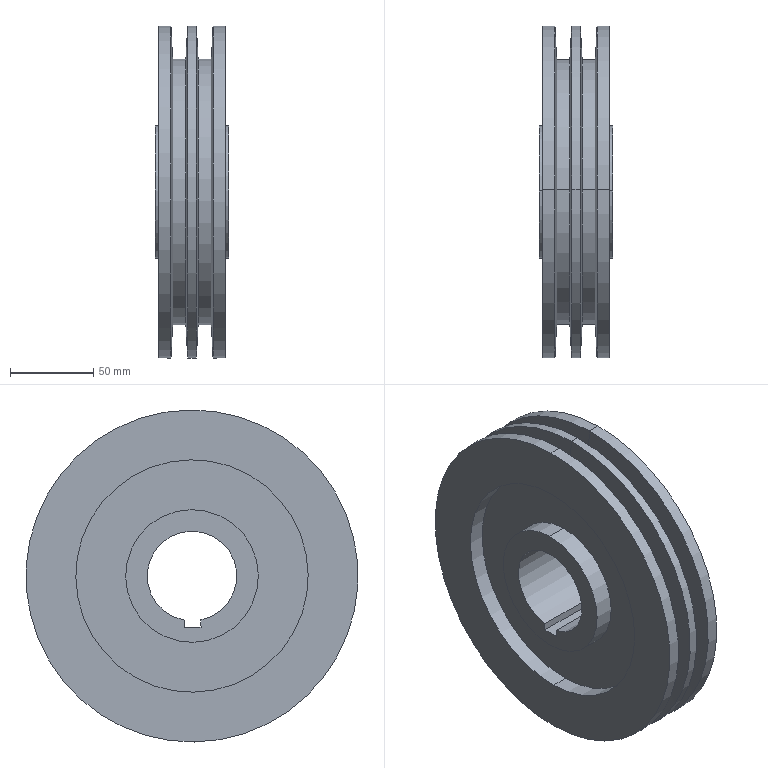Component | SolidWorks | Pulley1-1 | 1 solid | 37 faces | box 44 x 200 x 200 mm | volume 762387 mm3 | cylinder 20 | plane 9 | cone 8 | commonest cylinder face diameters 200 x6 160 x4 80 x4 140 x4 54 x2
build123d program:
from build123d import *

# Parameters (mm, degrees)
SKETCH1_5_R         = 100
SKETCH1_5_R_2       = 70
BOSS_EXTRUDE1_DEPTH = 20
SKETCH1_4_R         = 40
SKETCH1_4_R_2       = 27
BOSS_EXTRUDE2_DEPTH = 22
SKETCH1_5_2_R       = 70
SKETCH1_5_2_R_2     = 40
BOSS_EXTRUDE3_DEPTH = 10
SKETCH2_W           = 10
SKETCH2_H           = 8
CUT_EXTRUDE1_DEPTH  = 50


with BuildPart() as part:
    # Sketch1_5 → Boss-Extrude1 (new, symmetric)
    with BuildSketch(Plane(origin=(0, 0, 0), x_dir=(1, 0, 0), z_dir=(0, 1, 0))):
        with Locations(Location((0, 0, 0), (0, 0, 270))):
            Circle(SKETCH1_5_R)
        with Locations(Location((0, 0, 0), (0, 0, 270))):
            Circle(SKETCH1_5_R_2, mode=Mode.SUBTRACT)
    extrude(amount=BOSS_EXTRUDE1_DEPTH, both=True)



with BuildPart() as body_2:
    # Sketch1_4 → Boss-Extrude2 (new, symmetric)
    with BuildSketch(Plane(origin=(0, 0, 0), x_dir=(1, 0, 0), z_dir=(0, 1, 0))):
        with Locations(Location((0, 0, 0), (0, 0, 270))):
            Circle(SKETCH1_4_R)
        with Locations(Location((0, 0, 0), (0, 0, 270))):
            Circle(SKETCH1_4_R_2, mode=Mode.SUBTRACT)
    extrude(amount=BOSS_EXTRUDE2_DEPTH, both=True)


with BuildPart() as part_1:
    add(part.part)

    add(body_2.part)  # Boss-Extrude3 merges body 2
    # Sketch1_5 2 → Boss-Extrude3 (add, symmetric)
    with BuildSketch(Plane(origin=(0, 0, 0), x_dir=(1, 0, 0), z_dir=(0, 1, 0))):
        with Locations(Location((0, 0, 0), (0, 0, 270))):
            Circle(SKETCH1_5_2_R)
        with Locations(Location((0, 0, 0), (0, 0, 270))):
            Circle(SKETCH1_5_2_R_2, mode=Mode.SUBTRACT)
    extrude(amount=BOSS_EXTRUDE3_DEPTH, both=True)

    # Sketch2 → Cut-Extrude1 (cut)
    with BuildSketch(Plane.XZ.offset(22)):
        with Locations((0, 27)):
            Rectangle(SKETCH2_W, SKETCH2_H)
    extrude(amount=-CUT_EXTRUDE1_DEPTH, mode=Mode.SUBTRACT)

    # Sketch3 → Cut-Revolve1 (revolve, cut)
    with BuildSketch(Plane(origin=(0, 0, 0), x_dir=(0, 0, -1), z_dir=(1, 0, 0))):
        Polygon((-80, 7.676), (-80, 11.676), (-100, 12.676), (-100, 2.676), (-80, 3.676), align=None)
        Polygon((-80, -7.676), (-80, -11.676), (-100, -12.676), (-100, -2.676), (-80, -3.676), align=None)
    revolve(axis=Axis((0, 42.976, 0), (0, -1, 0)), mode=Mode.SUBTRACT)


solid = part_1.part

# Placed as in the assembly
solid = solid.moved(Location((141.571, -8.561, -165), (179.199, 0, -90)))
STEP:
#1=COLOUR_RGB('',0.7922,0.8196,0.9333);
#2=FILL_AREA_STYLE_COLOUR('',#1);
#3=FILL_AREA_STYLE('',(#2));
#4=SURFACE_STYLE_FILL_AREA(#3);
#5=SURFACE_SIDE_STYLE('',(#4));
#6=SURFACE_STYLE_USAGE(.BOTH.,#5);
#7=PRESENTATION_STYLE_ASSIGNMENT((#6));
#8=CARTESIAN_POINT('',(6.033,-0.3811,-9.645));
#9=VERTEX_POINT('',#8);
#10=CARTESIAN_POINT('',(6.033,-0.293,-3.347));
#11=VERTEX_POINT('',#10);
#12=CARTESIAN_POINT('',(6.033,-0.3371,-6.496));
#13=DIRECTION('',(-1.,-0.,-0.));
#14=DIRECTION('',(0.,-0.01398,-0.9999));
#15=AXIS2_PLACEMENT_3D('',#12,#13,#14);
#16=CIRCLE('',#15,3.15);
#17=EDGE_CURVE('',#9,#11,#16,.T.);
#18=ORIENTED_EDGE('',*,*,#17,.T.);
#19=CARTESIAN_POINT('',(5.718,-0.293,-3.347));
#20=VERTEX_POINT('',#19);
#21=CARTESIAN_POINT('',(3.882,-0.293,-3.347));
#22=DIRECTION('',(-1.,-0.,-0.));
#23=VECTOR('',#22,39.37);
#24=LINE('',#21,#23);
#25=EDGE_CURVE('',#11,#20,#24,.T.);
#26=ORIENTED_EDGE('',*,*,#25,.T.);
#27=CARTESIAN_POINT('',(5.718,-0.3811,-9.645));
#28=VERTEX_POINT('',#27);
#29=CARTESIAN_POINT('',(5.718,-0.3371,-6.496));
#30=DIRECTION('',(-1.,-0.,-0.));
#31=DIRECTION('',(0.,-0.01398,-0.9999));
#32=AXIS2_PLACEMENT_3D('',#29,#30,#31);
#33=CIRCLE('',#32,3.15);
#34=EDGE_CURVE('',#28,#20,#33,.T.);
#35=ORIENTED_EDGE('',*,*,#34,.F.);
#36=CARTESIAN_POINT('',(3.882,-0.3811,-9.645));
#37=DIRECTION('',(-1.,-0.,-0.));
#38=VECTOR('',#37,39.37);
#39=LINE('',#36,#38);
#40=EDGE_CURVE('',#9,#28,#39,.T.);
#41=ORIENTED_EDGE('',*,*,#40,.F.);
#42=EDGE_LOOP('',(#18,#26,#35,#41));
#43=FACE_OUTER_BOUND('',#42,.T.);
#44=CARTESIAN_POINT('',(3.882,-0.3371,-6.496));
#45=DIRECTION('',(-1.,-0.,-0.));
#46=DIRECTION('',(0.,-0.01398,-0.9999));
#47=AXIS2_PLACEMENT_3D('',#44,#45,#46);
#48=CYLINDRICAL_SURFACE('',#47,3.15);
#49=ADVANCED_FACE('',(#43),#48,.T.);
#50=ORIENTED_EDGE('',*,*,#17,.F.);
#51=CARTESIAN_POINT('',(6.073,-0.3921,-10.433));
#52=VERTEX_POINT('',#51);
#53=CARTESIAN_POINT('',(6.073,-0.3921,-10.433));
#54=DIRECTION('',(0.04994,-0.01396,-0.9987));
#55=VECTOR('',#54,39.37);
#56=LINE('',#53,#55);
#57=EDGE_CURVE('',#9,#52,#56,.T.);
#58=ORIENTED_EDGE('',*,*,#57,.T.);
#59=CARTESIAN_POINT('',(6.073,-0.282,-2.559));
#60=VERTEX_POINT('',#59);
#61=CARTESIAN_POINT('',(6.073,-0.3371,-6.496));
#62=DIRECTION('',(-1.,-0.,-0.));
#63=DIRECTION('',(0.,-0.01398,-0.9999));
#64=AXIS2_PLACEMENT_3D('',#61,#62,#63);
#65=CIRCLE('',#64,3.937);
#66=EDGE_CURVE('',#52,#60,#65,.T.);
#67=ORIENTED_EDGE('',*,*,#66,.T.);
#68=CARTESIAN_POINT('',(6.073,-0.282,-2.559));
#69=DIRECTION('',(0.04994,0.01396,0.9987));
#70=VECTOR('',#69,39.37);
#71=LINE('',#68,#70);
#72=EDGE_CURVE('',#11,#60,#71,.T.);
#73=ORIENTED_EDGE('',*,*,#72,.F.);
#74=EDGE_LOOP('',(#50,#58,#67,#73));
#75=FACE_OUTER_BOUND('',#74,.T.);
#76=CARTESIAN_POINT('',(6.073,-0.3371,-6.496));
#77=DIRECTION('',(1.,0.,0.));
#78=DIRECTION('',(0.,0.01398,0.9999));
#79=AXIS2_PLACEMENT_3D('',#76,#77,#78);
#80=CONICAL_SURFACE('',#79,3.937,1.521);
#81=ADVANCED_FACE('',(#75),#80,.T.);
#82=ORIENTED_EDGE('',*,*,#34,.T.);
#83=CARTESIAN_POINT('',(5.679,-0.282,-2.559));
#84=VERTEX_POINT('',#83);
#85=CARTESIAN_POINT('',(5.718,-0.293,-3.347));
#86=DIRECTION('',(-0.04994,0.01396,0.9987));
#87=VECTOR('',#86,39.37);
#88=LINE('',#85,#87);
#89=EDGE_CURVE('',#20,#84,#88,.T.);
#90=ORIENTED_EDGE('',*,*,#89,.T.);
#91=CARTESIAN_POINT('',(5.679,-0.3921,-10.433));
#92=VERTEX_POINT('',#91);
#93=CARTESIAN_POINT('',(5.679,-0.3371,-6.496));
#94=DIRECTION('',(-1.,-0.,-0.));
#95=DIRECTION('',(0.,-0.01398,-0.9999));
#96=AXIS2_PLACEMENT_3D('',#93,#94,#95);
#97=CIRCLE('',#96,3.937);
#98=EDGE_CURVE('',#92,#84,#97,.T.);
#99=ORIENTED_EDGE('',*,*,#98,.F.);
#100=CARTESIAN_POINT('',(5.718,-0.3811,-9.645));
#101=DIRECTION('',(-0.04994,-0.01396,-0.9987));
#102=VECTOR('',#101,39.37);
#103=LINE('',#100,#102);
#104=EDGE_CURVE('',#28,#92,#103,.T.);
#105=ORIENTED_EDGE('',*,*,#104,.F.);
#106=EDGE_LOOP('',(#82,#90,#99,#105));
#107=FACE_OUTER_BOUND('',#106,.T.);
#108=CARTESIAN_POINT('',(5.718,-0.3371,-6.496));
#109=DIRECTION('',(-1.,-0.,-0.));
#110=DIRECTION('',(0.,-0.01398,-0.9999));
#111=AXIS2_PLACEMENT_3D('',#108,#109,#110);
#112=CONICAL_SURFACE('',#111,3.15,1.521);
#113=ADVANCED_FACE('',(#107),#112,.T.);
#114=CARTESIAN_POINT('',(5.429,-0.3811,-9.645));
#115=VERTEX_POINT('',#114);
#116=CARTESIAN_POINT('',(5.429,-0.293,-3.347));
#117=VERTEX_POINT('',#116);
#118=CARTESIAN_POINT('',(5.429,-0.3371,-6.496));
#119=DIRECTION('',(-1.,-0.,-0.));
#120=DIRECTION('',(0.,-0.01398,-0.9999));
#121=AXIS2_PLACEMENT_3D('',#118,#119,#120);
#122=CIRCLE('',#121,3.15);
#123=EDGE_CURVE('',#115,#117,#122,.T.);
#124=ORIENTED_EDGE('',*,*,#123,.F.);
#125=CARTESIAN_POINT('',(5.468,-0.3921,-10.433));
#126=VERTEX_POINT('',#125);
#127=CARTESIAN_POINT('',(5.468,-0.3921,-10.433));
#128=DIRECTION('',(0.04994,-0.01396,-0.9987));
#129=VECTOR('',#128,39.37);
#130=LINE('',#127,#129);
#131=EDGE_CURVE('',#115,#126,#130,.T.);
#132=ORIENTED_EDGE('',*,*,#131,.T.);
#133=CARTESIAN_POINT('',(5.468,-0.282,-2.559));
#134=VERTEX_POINT('',#133);
#135=CARTESIAN_POINT('',(5.468,-0.3371,-6.496));
#136=DIRECTION('',(-1.,-0.,-0.));
#137=DIRECTION('',(0.,-0.01398,-0.9999));
#138=AXIS2_PLACEMENT_3D('',#135,#136,#137);
#139=CIRCLE('',#138,3.937);
#140=EDGE_CURVE('',#126,#134,#139,.T.);
#141=ORIENTED_EDGE('',*,*,#140,.T.);
#142=CARTESIAN_POINT('',(5.468,-0.282,-2.559));
#143=DIRECTION('',(0.04994,0.01396,0.9987));
#144=VECTOR('',#143,39.37);
#145=LINE('',#142,#144);
#146=EDGE_CURVE('',#117,#134,#145,.T.);
#147=ORIENTED_EDGE('',*,*,#146,.F.);
#148=EDGE_LOOP('',(#124,#132,#141,#147));
#149=FACE_OUTER_BOUND('',#148,.T.);
#150=CARTESIAN_POINT('',(5.468,-0.3371,-6.496));
#151=DIRECTION('',(1.,0.,0.));
#152=DIRECTION('',(0.,0.01398,0.9999));
#153=AXIS2_PLACEMENT_3D('',#150,#151,#152);
#154=CONICAL_SURFACE('',#153,3.937,1.521);
#155=ADVANCED_FACE('',(#149),#154,.T.);
#156=ORIENTED_EDGE('',*,*,#123,.T.);
#157=CARTESIAN_POINT('',(5.114,-0.293,-3.347));
#158=VERTEX_POINT('',#157);
#159=CARTESIAN_POINT('',(3.882,-0.293,-3.347));
#160=DIRECTION('',(-1.,-0.,-0.));
#161=VECTOR('',#160,39.37);
#162=LINE('',#159,#161);
#163=EDGE_CURVE('',#117,#158,#162,.T.);
#164=ORIENTED_EDGE('',*,*,#163,.T.);
#165=CARTESIAN_POINT('',(5.114,-0.3811,-9.645));
#166=VERTEX_POINT('',#165);
#167=CARTESIAN_POINT('',(5.114,-0.3371,-6.496));
#168=DIRECTION('',(-1.,-0.,-0.));
#169=DIRECTION('',(0.,-0.01398,-0.9999));
#170=AXIS2_PLACEMENT_3D('',#167,#168,#169);
#171=CIRCLE('',#170,3.15);
#172=EDGE_CURVE('',#166,#158,#171,.T.);
#173=ORIENTED_EDGE('',*,*,#172,.F.);
#174=CARTESIAN_POINT('',(3.882,-0.3811,-9.645));
#175=DIRECTION('',(-1.,-0.,-0.));
#176=VECTOR('',#175,39.37);
#177=LINE('',#174,#176);
#178=EDGE_CURVE('',#115,#166,#177,.T.);
#179=ORIENTED_EDGE('',*,*,#178,.F.);
#180=EDGE_LOOP('',(#156,#164,#173,#179));
#181=FACE_OUTER_BOUND('',#180,.T.);
#182=CARTESIAN_POINT('',(3.882,-0.3371,-6.496));
#183=DIRECTION('',(-1.,-0.,-0.));
#184=DIRECTION('',(0.,-0.01398,-0.9999));
#185=AXIS2_PLACEMENT_3D('',#182,#183,#184);
#186=CYLINDRICAL_SURFACE('',#185,3.15);
#187=ADVANCED_FACE('',(#181),#186,.T.);
#188=ORIENTED_EDGE('',*,*,#172,.T.);
#189=CARTESIAN_POINT('',(5.075,-0.282,-2.559));
#190=VERTEX_POINT('',#189);
#191=CARTESIAN_POINT('',(5.114,-0.293,-3.347));
#192=DIRECTION('',(-0.04994,0.01396,0.9987));
#193=VECTOR('',#192,39.37);
#194=LINE('',#191,#193);
#195=EDGE_CURVE('',#158,#190,#194,.T.);
#196=ORIENTED_EDGE('',*,*,#195,.T.);
#197=CARTESIAN_POINT('',(5.075,-0.3921,-10.433));
#198=VERTEX_POINT('',#197);
#199=CARTESIAN_POINT('',(5.075,-0.3371,-6.496));
#200=DIRECTION('',(-1.,-0.,-0.));
#201=DIRECTION('',(0.,-0.01398,-0.9999));
#202=AXIS2_PLACEMENT_3D('',#199,#200,#201);
#203=CIRCLE('',#202,3.937);
#204=EDGE_CURVE('',#198,#190,#203,.T.);
#205=ORIENTED_EDGE('',*,*,#204,.F.);
#206=CARTESIAN_POINT('',(5.114,-0.3811,-9.645));
#207=DIRECTION('',(-0.04994,-0.01396,-0.9987));
#208=VECTOR('',#207,39.37);
#209=LINE('',#206,#208);
#210=EDGE_CURVE('',#166,#198,#209,.T.);
#211=ORIENTED_EDGE('',*,*,#210,.F.);
#212=EDGE_LOOP('',(#188,#196,#205,#211));
#213=FACE_OUTER_BOUND('',#212,.T.);
#214=CARTESIAN_POINT('',(5.114,-0.3371,-6.496));
#215=DIRECTION('',(-1.,-0.,-0.));
#216=DIRECTION('',(0.,-0.01398,-0.9999));
#217=AXIS2_PLACEMENT_3D('',#214,#215,#216);
#218=CONICAL_SURFACE('',#217,3.15,1.521);
#219=ADVANCED_FACE('',(#213),#218,.T.);
#220=CARTESIAN_POINT('',(4.708,-0.3591,-8.071));
#221=VERTEX_POINT('',#220);
#222=CARTESIAN_POINT('',(4.708,-0.315,-4.921));
#223=VERTEX_POINT('',#222);
#224=CARTESIAN_POINT('',(4.708,-0.3371,-6.496));
#225=DIRECTION('',(-1.,-0.,-0.));
#226=DIRECTION('',(0.,-0.01398,-0.9999));
#227=AXIS2_PLACEMENT_3D('',#224,#225,#226);
#228=CIRCLE('',#227,1.575);
#229=EDGE_CURVE('',#221,#223,#228,.T.);
#230=ORIENTED_EDGE('',*,*,#229,.F.);
#231=CARTESIAN_POINT('',(5.18,-0.3591,-8.071));
#232=VERTEX_POINT('',#231);
#233=CARTESIAN_POINT('',(4.708,-0.3591,-8.071));
#234=DIRECTION('',(1.,0.,0.));
#235=VECTOR('',#234,39.37);
#236=LINE('',#233,#235);
#237=EDGE_CURVE('',#221,#232,#236,.T.);
#238=ORIENTED_EDGE('',*,*,#237,.T.);
#239=CARTESIAN_POINT('',(5.18,-0.315,-4.921));
#240=VERTEX_POINT('',#239);
#241=CARTESIAN_POINT('',(5.18,-0.3371,-6.496));
#242=DIRECTION('',(-1.,-0.,-0.));
#243=DIRECTION('',(0.,-0.01398,-0.9999));
#244=AXIS2_PLACEMENT_3D('',#241,#242,#243);
#245=CIRCLE('',#244,1.575);
#246=EDGE_CURVE('',#232,#240,#245,.T.);
#247=ORIENTED_EDGE('',*,*,#246,.T.);
#248=CARTESIAN_POINT('',(4.708,-0.315,-4.921));
#249=DIRECTION('',(1.,0.,0.));
#250=VECTOR('',#249,39.37);
#251=LINE('',#248,#250);
#252=EDGE_CURVE('',#223,#240,#251,.T.);
#253=ORIENTED_EDGE('',*,*,#252,.F.);
#254=EDGE_LOOP('',(#230,#238,#247,#253));
#255=FACE_OUTER_BOUND('',#254,.T.);
#256=CARTESIAN_POINT('',(4.708,-0.3371,-6.496));
#257=DIRECTION('',(1.,0.,0.));
#258=DIRECTION('',(0.,0.01398,0.9999));
#259=AXIS2_PLACEMENT_3D('',#256,#257,#258);
#260=CYLINDRICAL_SURFACE('',#259,1.575);
#261=ADVANCED_FACE('',(#255),#260,.T.);
#262=CARTESIAN_POINT('',(4.708,-0.5485,-7.538));
#263=VERTEX_POINT('',#262);
#264=CARTESIAN_POINT('',(4.708,-0.3222,-5.433));
#265=VERTEX_POINT('',#264);
#266=CARTESIAN_POINT('',(4.708,-0.3371,-6.496));
#267=DIRECTION('',(-1.,-0.,-0.));
#268=DIRECTION('',(0.,-0.01398,-0.9999));
#269=AXIS2_PLACEMENT_3D('',#266,#267,#268);
#270=CIRCLE('',#269,1.063);
#271=EDGE_CURVE('',#263,#265,#270,.T.);
#272=ORIENTED_EDGE('',*,*,#271,.T.);
#273=CARTESIAN_POINT('',(6.44,-0.3222,-5.433));
#274=VERTEX_POINT('',#273);
#275=CARTESIAN_POINT('',(4.708,-0.3222,-5.433));
#276=DIRECTION('',(1.,0.,0.));
#277=VECTOR('',#276,39.37);
#278=LINE('',#275,#277);
#279=EDGE_CURVE('',#265,#274,#278,.T.);
#280=ORIENTED_EDGE('',*,*,#279,.T.);
#281=CARTESIAN_POINT('',(6.44,-0.5485,-7.538));
#282=VERTEX_POINT('',#281);
#283=CARTESIAN_POINT('',(6.44,-0.3371,-6.496));
#284=DIRECTION('',(-1.,-0.,-0.));
#285=DIRECTION('',(0.,-0.01398,-0.9999));
#286=AXIS2_PLACEMENT_3D('',#283,#284,#285);
#287=CIRCLE('',#286,1.063);
#288=EDGE_CURVE('',#282,#274,#287,.T.);
#289=ORIENTED_EDGE('',*,*,#288,.F.);
#290=CARTESIAN_POINT('',(4.708,-0.5485,-7.538));
#291=DIRECTION('',(1.,0.,0.));
#292=VECTOR('',#291,39.37);
#293=LINE('',#290,#292);
#294=EDGE_CURVE('',#263,#282,#293,.T.);
#295=ORIENTED_EDGE('',*,*,#294,.F.);
#296=EDGE_LOOP('',(#272,#280,#289,#295));
#297=FACE_OUTER_BOUND('',#296,.T.);
#298=CARTESIAN_POINT('',(4.708,-0.3371,-6.496));
#299=DIRECTION('',(1.,0.,0.));
#300=DIRECTION('',(0.,0.01398,0.9999));
#301=AXIS2_PLACEMENT_3D('',#298,#299,#300);
#302=CYLINDRICAL_SURFACE('',#301,1.063);
#303=ADVANCED_FACE('',(#297),#302,.F.);
#304=CARTESIAN_POINT('',(5.967,-0.315,-4.921));
#305=VERTEX_POINT('',#304);
#306=CARTESIAN_POINT('',(5.967,-0.3591,-8.071));
#307=VERTEX_POINT('',#306);
#308=CARTESIAN_POINT('',(5.967,-0.3371,-6.496));
#309=DIRECTION('',(1.,0.,0.));
#310=DIRECTION('',(0.,-0.01398,-0.9999));
#311=AXIS2_PLACEMENT_3D('',#308,#309,#310);
#312=CIRCLE('',#311,1.575);
#313=EDGE_CURVE('',#305,#307,#312,.T.);
#314=ORIENTED_EDGE('',*,*,#313,.T.);
#315=CARTESIAN_POINT('',(6.44,-0.3591,-8.071));
#316=VERTEX_POINT('',#315);
#317=CARTESIAN_POINT('',(4.708,-0.3591,-8.071));
#318=DIRECTION('',(1.,0.,0.));
#319=VECTOR('',#318,39.37);
#320=LINE('',#317,#319);
#321=EDGE_CURVE('',#307,#316,#320,.T.);
#322=ORIENTED_EDGE('',*,*,#321,.T.);
#323=CARTESIAN_POINT('',(6.44,-0.315,-4.921));
#324=VERTEX_POINT('',#323);
#325=CARTESIAN_POINT('',(6.44,-0.3371,-6.496));
#326=DIRECTION('',(-1.,-0.,-0.));
#327=DIRECTION('',(0.,-0.01398,-0.9999));
#328=AXIS2_PLACEMENT_3D('',#325,#326,#327);
#329=CIRCLE('',#328,1.575);
#330=EDGE_CURVE('',#316,#324,#329,.T.);
#331=ORIENTED_EDGE('',*,*,#330,.T.);
#332=CARTESIAN_POINT('',(4.708,-0.315,-4.921));
#333=DIRECTION('',(1.,0.,0.));
#334=VECTOR('',#333,39.37);
#335=LINE('',#332,#334);
#336=EDGE_CURVE('',#305,#324,#335,.T.);
#337=ORIENTED_EDGE('',*,*,#336,.F.);
#338=EDGE_LOOP('',(#314,#322,#331,#337));
#339=FACE_OUTER_BOUND('',#338,.T.);
#340=CARTESIAN_POINT('',(4.708,-0.3371,-6.496));
#341=DIRECTION('',(1.,0.,0.));
#342=DIRECTION('',(0.,0.01398,0.9999));
#343=AXIS2_PLACEMENT_3D('',#340,#341,#342);
#344=CYLINDRICAL_SURFACE('',#343,1.575);
#345=ADVANCED_FACE('',(#339),#344,.T.);
#346=ORIENTED_EDGE('',*,*,#66,.F.);
#347=CARTESIAN_POINT('',(6.361,-0.3921,-10.433));
#348=VERTEX_POINT('',#347);
#349=CARTESIAN_POINT('',(4.786,-0.3921,-10.433));
#350=DIRECTION('',(1.,0.,0.));
#351=VECTOR('',#350,39.37);
#352=LINE('',#349,#351);
#353=EDGE_CURVE('',#52,#348,#352,.T.);
#354=ORIENTED_EDGE('',*,*,#353,.T.);
#355=CARTESIAN_POINT('',(6.361,-0.282,-2.559));
#356=VERTEX_POINT('',#355);
#357=CARTESIAN_POINT('',(6.361,-0.3371,-6.496));
#358=DIRECTION('',(-1.,-0.,-0.));
#359=DIRECTION('',(0.,-0.01398,-0.9999));
#360=AXIS2_PLACEMENT_3D('',#357,#358,#359);
#361=CIRCLE('',#360,3.937);
#362=EDGE_CURVE('',#348,#356,#361,.T.);
#363=ORIENTED_EDGE('',*,*,#362,.T.);
#364=CARTESIAN_POINT('',(4.786,-0.282,-2.559));
#365=DIRECTION('',(1.,0.,0.));
#366=VECTOR('',#365,39.37);
#367=LINE('',#364,#366);
#368=EDGE_CURVE('',#60,#356,#367,.T.);
#369=ORIENTED_EDGE('',*,*,#368,.F.);
#370=EDGE_LOOP('',(#346,#354,#363,#369));
#371=FACE_OUTER_BOUND('',#370,.T.);
#372=CARTESIAN_POINT('',(4.786,-0.3371,-6.496));
#373=DIRECTION('',(1.,0.,0.));
#374=DIRECTION('',(-0.,0.01398,0.9999));
#375=AXIS2_PLACEMENT_3D('',#372,#373,#374);
#376=CYLINDRICAL_SURFACE('',#375,3.937);
#377=ADVANCED_FACE('',(#371),#376,.T.);
#378=CARTESIAN_POINT('',(4.786,-0.2985,-3.74));
#379=VERTEX_POINT('',#378);
#380=CARTESIAN_POINT('',(4.786,-0.3756,-9.252));
#381=VERTEX_POINT('',#380);
#382=CARTESIAN_POINT('',(4.786,-0.3371,-6.496));
#383=DIRECTION('',(-1.,-0.,-0.));
#384=DIRECTION('',(0.,-0.01398,-0.9999));
#385=AXIS2_PLACEMENT_3D('',#382,#383,#384);
#386=CIRCLE('',#385,2.756);
#387=EDGE_CURVE('',#379,#381,#386,.T.);
#388=ORIENTED_EDGE('',*,*,#387,.T.);
#389=CARTESIAN_POINT('',(5.18,-0.3756,-9.252));
#390=VERTEX_POINT('',#389);
#391=CARTESIAN_POINT('',(4.786,-0.3756,-9.252));
#392=DIRECTION('',(1.,0.,0.));
#393=VECTOR('',#392,39.37);
#394=LINE('',#391,#393);
#395=EDGE_CURVE('',#381,#390,#394,.T.);
#396=ORIENTED_EDGE('',*,*,#395,.T.);
#397=CARTESIAN_POINT('',(5.18,-0.2985,-3.74));
#398=VERTEX_POINT('',#397);
#399=CARTESIAN_POINT('',(5.18,-0.3371,-6.496));
#400=DIRECTION('',(-1.,-0.,-0.));
#401=DIRECTION('',(0.,-0.01398,-0.9999));
#402=AXIS2_PLACEMENT_3D('',#399,#400,#401);
#403=CIRCLE('',#402,2.756);
#404=EDGE_CURVE('',#398,#390,#403,.T.);
#405=ORIENTED_EDGE('',*,*,#404,.F.);
#406=CARTESIAN_POINT('',(4.786,-0.2985,-3.74));
#407=DIRECTION('',(1.,0.,0.));
#408=VECTOR('',#407,39.37);
#409=LINE('',#406,#408);
#410=EDGE_CURVE('',#379,#398,#409,.T.);
#411=ORIENTED_EDGE('',*,*,#410,.F.);
#412=EDGE_LOOP('',(#388,#396,#405,#411));
#413=FACE_OUTER_BOUND('',#412,.T.);
#414=CARTESIAN_POINT('',(4.786,-0.3371,-6.496));
#415=DIRECTION('',(1.,0.,0.));
#416=DIRECTION('',(0.,0.01398,0.9999));
#417=AXIS2_PLACEMENT_3D('',#414,#415,#416);
#418=CYLINDRICAL_SURFACE('',#417,2.756);
#419=ADVANCED_FACE('',(#413),#418,.F.);
#420=CARTESIAN_POINT('',(5.967,-0.2985,-3.74));
#421=VERTEX_POINT('',#420);
#422=CARTESIAN_POINT('',(5.967,-0.3756,-9.252));
#423=VERTEX_POINT('',#422);
#424=CARTESIAN_POINT('',(5.967,-0.3371,-6.496));
#425=DIRECTION('',(-1.,-0.,-0.));
#426=DIRECTION('',(0.,-0.01398,-0.9999));
#427=AXIS2_PLACEMENT_3D('',#424,#425,#426);
#428=CIRCLE('',#427,2.756);
#429=EDGE_CURVE('',#421,#423,#428,.T.);
#430=ORIENTED_EDGE('',*,*,#429,.T.);
#431=CARTESIAN_POINT('',(6.361,-0.3756,-9.252));
#432=VERTEX_POINT('',#431);
#433=CARTESIAN_POINT('',(4.786,-0.3756,-9.252));
#434=DIRECTION('',(1.,0.,0.));
#435=VECTOR('',#434,39.37);
#436=LINE('',#433,#435);
#437=EDGE_CURVE('',#423,#432,#436,.T.);
#438=ORIENTED_EDGE('',*,*,#437,.T.);
#439=CARTESIAN_POINT('',(6.361,-0.2985,-3.74));
#440=VERTEX_POINT('',#439);
#441=CARTESIAN_POINT('',(6.361,-0.3371,-6.496));
#442=DIRECTION('',(-1.,-0.,-0.));
#443=DIRECTION('',(0.,-0.01398,-0.9999));
#444=AXIS2_PLACEMENT_3D('',#441,#442,#443);
#445=CIRCLE('',#444,2.756);
#446=EDGE_CURVE('',#440,#432,#445,.T.);
#447=ORIENTED_EDGE('',*,*,#446,.F.);
#448=CARTESIAN_POINT('',(4.786,-0.2985,-3.74));
#449=DIRECTION('',(1.,0.,0.));
#450=VECTOR('',#449,39.37);
#451=LINE('',#448,#450);
#452=EDGE_CURVE('',#421,#440,#451,.T.);
#453=ORIENTED_EDGE('',*,*,#452,.F.);
#454=EDGE_LOOP('',(#430,#438,#447,#453));
#455=FACE_OUTER_BOUND('',#454,.T.);
#456=CARTESIAN_POINT('',(4.786,-0.3371,-6.496));
#457=DIRECTION('',(1.,0.,0.));
#458=DIRECTION('',(0.,0.01398,0.9999));
#459=AXIS2_PLACEMENT_3D('',#456,#457,#458);
#460=CYLINDRICAL_SURFACE('',#459,2.756);
#461=ADVANCED_FACE('',(#455),#460,.F.);
#462=CARTESIAN_POINT('',(4.786,-0.3921,-10.433));
#463=VERTEX_POINT('',#462);
#464=CARTESIAN_POINT('',(4.786,-0.282,-2.559));
#465=VERTEX_POINT('',#464);
#466=CARTESIAN_POINT('',(4.786,-0.3371,-6.496));
#467=DIRECTION('',(-1.,-0.,-0.));
#468=DIRECTION('',(0.,-0.01398,-0.9999));
#469=AXIS2_PLACEMENT_3D('',#466,#467,#468);
#470=CIRCLE('',#469,3.937);
#471=EDGE_CURVE('',#463,#465,#470,.T.);
#472=ORIENTED_EDGE('',*,*,#471,.F.);
#473=CARTESIAN_POINT('',(4.786,-0.3921,-10.433));
#474=DIRECTION('',(1.,0.,0.));
#475=VECTOR('',#474,39.37);
#476=LINE('',#473,#475);
#477=EDGE_CURVE('',#463,#198,#476,.T.);
#478=ORIENTED_EDGE('',*,*,#477,.T.);
#479=ORIENTED_EDGE('',*,*,#204,.T.);
#480=CARTESIAN_POINT('',(4.786,-0.282,-2.559));
#481=DIRECTION('',(1.,0.,0.));
#482=VECTOR('',#481,39.37);
#483=LINE('',#480,#482);
#484=EDGE_CURVE('',#465,#190,#483,.T.);
#485=ORIENTED_EDGE('',*,*,#484,.F.);
#486=EDGE_LOOP('',(#472,#478,#479,#485));
#487=FACE_OUTER_BOUND('',#486,.T.);
#488=CARTESIAN_POINT('',(4.786,-0.3371,-6.496));
#489=DIRECTION('',(1.,0.,0.));
#490=DIRECTION('',(-0.,0.01398,0.9999));
#491=AXIS2_PLACEMENT_3D('',#488,#489,#490);
#492=CYLINDRICAL_SURFACE('',#491,3.937);
#493=ADVANCED_FACE('',(#487),#492,.T.);
#494=ORIENTED_EDGE('',*,*,#140,.F.);
#495=CARTESIAN_POINT('',(4.786,-0.3921,-10.433));
#496=DIRECTION('',(1.,0.,0.));
#497=VECTOR('',#496,39.37);
#498=LINE('',#495,#497);
#499=EDGE_CURVE('',#126,#92,#498,.T.);
#500=ORIENTED_EDGE('',*,*,#499,.T.);
#501=ORIENTED_EDGE('',*,*,#98,.T.);
#502=CARTESIAN_POINT('',(4.786,-0.282,-2.559));
#503=DIRECTION('',(1.,0.,0.));
#504=VECTOR('',#503,39.37);
#505=LINE('',#502,#504);
#506=EDGE_CURVE('',#134,#84,#505,.T.);
#507=ORIENTED_EDGE('',*,*,#506,.F.);
#508=EDGE_LOOP('',(#494,#500,#501,#507));
#509=FACE_OUTER_BOUND('',#508,.T.);
#510=CARTESIAN_POINT('',(4.786,-0.3371,-6.496));
#511=DIRECTION('',(1.,0.,0.));
#512=DIRECTION('',(-0.,0.01398,0.9999));
#513=AXIS2_PLACEMENT_3D('',#510,#511,#512);
#514=CYLINDRICAL_SURFACE('',#513,3.937);
#515=ADVANCED_FACE('',(#509),#514,.T.);
#516=ORIENTED_EDGE('',*,*,#499,.F.);
#517=CARTESIAN_POINT('',(5.468,-0.3371,-6.496));
#518=DIRECTION('',(-1.,-0.,-0.));
#519=DIRECTION('',(0.,-0.01398,-0.9999));
#520=AXIS2_PLACEMENT_3D('',#517,#518,#519);
#521=CIRCLE('',#520,3.937);
#522=EDGE_CURVE('',#134,#126,#521,.T.);
#523=ORIENTED_EDGE('',*,*,#522,.F.);
#524=ORIENTED_EDGE('',*,*,#506,.T.);
#525=CARTESIAN_POINT('',(5.679,-0.3371,-6.496));
#526=DIRECTION('',(-1.,-0.,-0.));
#527=DIRECTION('',(0.,-0.01398,-0.9999));
#528=AXIS2_PLACEMENT_3D('',#525,#526,#527);
#529=CIRCLE('',#528,3.937);
#530=EDGE_CURVE('',#84,#92,#529,.T.);
#531=ORIENTED_EDGE('',*,*,#530,.T.);
#532=EDGE_LOOP('',(#516,#523,#524,#531));
#533=FACE_OUTER_BOUND('',#532,.T.);
#534=CARTESIAN_POINT('',(4.786,-0.3371,-6.496));
#535=DIRECTION('',(1.,0.,0.));
#536=DIRECTION('',(-0.,0.01398,0.9999));
#537=AXIS2_PLACEMENT_3D('',#534,#535,#536);
#538=CYLINDRICAL_SURFACE('',#537,3.937);
#539=ADVANCED_FACE('',(#533),#538,.T.);
#540=ORIENTED_EDGE('',*,*,#477,.F.);
#541=CARTESIAN_POINT('',(4.786,-0.3371,-6.496));
#542=DIRECTION('',(-1.,-0.,-0.));
#543=DIRECTION('',(0.,-0.01398,-0.9999));
#544=AXIS2_PLACEMENT_3D('',#541,#542,#543);
#545=CIRCLE('',#544,3.937);
#546=EDGE_CURVE('',#465,#463,#545,.T.);
#547=ORIENTED_EDGE('',*,*,#546,.F.);
#548=ORIENTED_EDGE('',*,*,#484,.T.);
#549=CARTESIAN_POINT('',(5.075,-0.3371,-6.496));
#550=DIRECTION('',(-1.,-0.,-0.));
#551=DIRECTION('',(0.,-0.01398,-0.9999));
#552=AXIS2_PLACEMENT_3D('',#549,#550,#551);
#553=CIRCLE('',#552,3.937);
#554=EDGE_CURVE('',#190,#198,#553,.T.);
#555=ORIENTED_EDGE('',*,*,#554,.T.);
#556=EDGE_LOOP('',(#540,#547,#548,#555));
#557=FACE_OUTER_BOUND('',#556,.T.);
#558=CARTESIAN_POINT('',(4.786,-0.3371,-6.496));
#559=DIRECTION('',(1.,0.,0.));
#560=DIRECTION('',(-0.,0.01398,0.9999));
#561=AXIS2_PLACEMENT_3D('',#558,#559,#560);
#562=CYLINDRICAL_SURFACE('',#561,3.937);
#563=ADVANCED_FACE('',(#557),#562,.T.);
#564=ORIENTED_EDGE('',*,*,#437,.F.);
#565=CARTESIAN_POINT('',(5.967,-0.3371,-6.496));
#566=DIRECTION('',(-1.,-0.,-0.));
#567=DIRECTION('',(0.,-0.01398,-0.9999));
#568=AXIS2_PLACEMENT_3D('',#565,#566,#567);
#569=CIRCLE('',#568,2.756);
#570=EDGE_CURVE('',#423,#421,#569,.T.);
#571=ORIENTED_EDGE('',*,*,#570,.T.);
#572=ORIENTED_EDGE('',*,*,#452,.T.);
#573=CARTESIAN_POINT('',(6.361,-0.3371,-6.496));
#574=DIRECTION('',(-1.,-0.,-0.));
#575=DIRECTION('',(0.,-0.01398,-0.9999));
#576=AXIS2_PLACEMENT_3D('',#573,#574,#575);
#577=CIRCLE('',#576,2.756);
#578=EDGE_CURVE('',#432,#440,#577,.T.);
#579=ORIENTED_EDGE('',*,*,#578,.F.);
#580=EDGE_LOOP('',(#564,#571,#572,#579));
#581=FACE_OUTER_BOUND('',#580,.T.);
#582=CARTESIAN_POINT('',(4.786,-0.3371,-6.496));
#583=DIRECTION('',(1.,0.,0.));
#584=DIRECTION('',(0.,0.01398,0.9999));
#585=AXIS2_PLACEMENT_3D('',#582,#583,#584);
#586=CYLINDRICAL_SURFACE('',#585,2.756);
#587=ADVANCED_FACE('',(#581),#586,.F.);
#588=ORIENTED_EDGE('',*,*,#395,.F.);
#589=CARTESIAN_POINT('',(4.786,-0.3371,-6.496));
#590=DIRECTION('',(-1.,-0.,-0.));
#591=DIRECTION('',(0.,-0.01398,-0.9999));
#592=AXIS2_PLACEMENT_3D('',#589,#590,#591);
#593=CIRCLE('',#592,2.756);
#594=EDGE_CURVE('',#381,#379,#593,.T.);
#595=ORIENTED_EDGE('',*,*,#594,.T.);
#596=ORIENTED_EDGE('',*,*,#410,.T.);
#597=CARTESIAN_POINT('',(5.18,-0.3371,-6.496));
#598=DIRECTION('',(-1.,-0.,-0.));
#599=DIRECTION('',(0.,-0.01398,-0.9999));
#600=AXIS2_PLACEMENT_3D('',#597,#598,#599);
#601=CIRCLE('',#600,2.756);
#602=EDGE_CURVE('',#390,#398,#601,.T.);
#603=ORIENTED_EDGE('',*,*,#602,.F.);
#604=EDGE_LOOP('',(#588,#595,#596,#603));
#605=FACE_OUTER_BOUND('',#604,.T.);
#606=CARTESIAN_POINT('',(4.786,-0.3371,-6.496));
#607=DIRECTION('',(1.,0.,0.));
#608=DIRECTION('',(0.,0.01398,0.9999));
#609=AXIS2_PLACEMENT_3D('',#606,#607,#608);
#610=CYLINDRICAL_SURFACE('',#609,2.756);
#611=ADVANCED_FACE('',(#605),#610,.F.);
#612=ORIENTED_EDGE('',*,*,#353,.F.);
#613=CARTESIAN_POINT('',(6.073,-0.3371,-6.496));
#614=DIRECTION('',(-1.,-0.,-0.));
#615=DIRECTION('',(0.,-0.01398,-0.9999));
#616=AXIS2_PLACEMENT_3D('',#613,#614,#615);
#617=CIRCLE('',#616,3.937);
#618=EDGE_CURVE('',#60,#52,#617,.T.);
#619=ORIENTED_EDGE('',*,*,#618,.F.);
#620=ORIENTED_EDGE('',*,*,#368,.T.);
#621=CARTESIAN_POINT('',(6.361,-0.3371,-6.496));
#622=DIRECTION('',(-1.,-0.,-0.));
#623=DIRECTION('',(0.,-0.01398,-0.9999));
#624=AXIS2_PLACEMENT_3D('',#621,#622,#623);
#625=CIRCLE('',#624,3.937);
#626=EDGE_CURVE('',#356,#348,#625,.T.);
#627=ORIENTED_EDGE('',*,*,#626,.T.);
#628=EDGE_LOOP('',(#612,#619,#620,#627));
#629=FACE_OUTER_BOUND('',#628,.T.);
#630=CARTESIAN_POINT('',(4.786,-0.3371,-6.496));
#631=DIRECTION('',(1.,0.,0.));
#632=DIRECTION('',(-0.,0.01398,0.9999));
#633=AXIS2_PLACEMENT_3D('',#630,#631,#632);
#634=CYLINDRICAL_SURFACE('',#633,3.937);
#635=ADVANCED_FACE('',(#629),#634,.T.);
#636=ORIENTED_EDGE('',*,*,#387,.F.);
#637=ORIENTED_EDGE('',*,*,#594,.F.);
#638=EDGE_LOOP('',(#636,#637));
#639=FACE_BOUND('',#638,.T.);
#640=ORIENTED_EDGE('',*,*,#546,.T.);
#641=ORIENTED_EDGE('',*,*,#471,.T.);
#642=EDGE_LOOP('',(#640,#641));
#643=FACE_OUTER_BOUND('',#642,.T.);
#644=CARTESIAN_POINT('',(4.786,8.329,-6.617));
#645=DIRECTION('',(-1.,-0.,-0.));
#646=DIRECTION('',(0.,-0.01398,-0.9999));
#647=AXIS2_PLACEMENT_3D('',#644,#645,#646);
#648=PLANE('',#647);
#649=ADVANCED_FACE('',(#639,#643),#648,.T.);
#650=ORIENTED_EDGE('',*,*,#446,.T.);
#651=ORIENTED_EDGE('',*,*,#578,.T.);
#652=EDGE_LOOP('',(#650,#651));
#653=FACE_BOUND('',#652,.T.);
#654=ORIENTED_EDGE('',*,*,#626,.F.);
#655=ORIENTED_EDGE('',*,*,#362,.F.);
#656=EDGE_LOOP('',(#654,#655));
#657=FACE_OUTER_BOUND('',#656,.T.);
#658=CARTESIAN_POINT('',(6.361,8.329,-6.617));
#659=DIRECTION('',(-1.,-0.,-0.));
#660=DIRECTION('',(0.,-0.01398,-0.9999));
#661=AXIS2_PLACEMENT_3D('',#658,#659,#660);
#662=PLANE('',#661);
#663=ADVANCED_FACE('',(#653,#657),#662,.F.);
#664=CARTESIAN_POINT('',(5.18,-0.3371,-6.496));
#665=DIRECTION('',(-1.,-0.,-0.));
#666=DIRECTION('',(0.,-0.01398,-0.9999));
#667=AXIS2_PLACEMENT_3D('',#664,#665,#666);
#668=CIRCLE('',#667,1.575);
#669=EDGE_CURVE('',#240,#232,#668,.T.);
#670=ORIENTED_EDGE('',*,*,#669,.F.);
#671=ORIENTED_EDGE('',*,*,#246,.F.);
#672=EDGE_LOOP('',(#670,#671));
#673=FACE_BOUND('',#672,.T.);
#674=ORIENTED_EDGE('',*,*,#404,.T.);
#675=ORIENTED_EDGE('',*,*,#602,.T.);
#676=EDGE_LOOP('',(#674,#675));
#677=FACE_OUTER_BOUND('',#676,.T.);
#678=CARTESIAN_POINT('',(5.18,8.329,-6.617));
#679=DIRECTION('',(-1.,-0.,-0.));
#680=DIRECTION('',(0.,-0.01398,-0.9999));
#681=AXIS2_PLACEMENT_3D('',#678,#679,#680);
#682=PLANE('',#681);
#683=ADVANCED_FACE('',(#673,#677),#682,.T.);
#684=ORIENTED_EDGE('',*,*,#313,.F.);
#685=CARTESIAN_POINT('',(5.967,-0.3371,-6.496));
#686=DIRECTION('',(1.,0.,0.));
#687=DIRECTION('',(0.,-0.01398,-0.9999));
#688=AXIS2_PLACEMENT_3D('',#685,#686,#687);
#689=CIRCLE('',#688,1.575);
#690=EDGE_CURVE('',#307,#305,#689,.T.);
#691=ORIENTED_EDGE('',*,*,#690,.F.);
#692=EDGE_LOOP('',(#684,#691));
#693=FACE_BOUND('',#692,.T.);
#694=ORIENTED_EDGE('',*,*,#429,.F.);
#695=ORIENTED_EDGE('',*,*,#570,.F.);
#696=EDGE_LOOP('',(#694,#695));
#697=FACE_OUTER_BOUND('',#696,.T.);
#698=CARTESIAN_POINT('',(5.967,8.329,-6.617));
#699=DIRECTION('',(-1.,-0.,-0.));
#700=DIRECTION('',(0.,-0.01398,-0.9999));
#701=AXIS2_PLACEMENT_3D('',#698,#699,#700);
#702=PLANE('',#701);
#703=ADVANCED_FACE('',(#693,#697),#702,.F.);
#704=ORIENTED_EDGE('',*,*,#321,.F.);
#705=ORIENTED_EDGE('',*,*,#690,.T.);
#706=ORIENTED_EDGE('',*,*,#336,.T.);
#707=CARTESIAN_POINT('',(6.44,-0.3371,-6.496));
#708=DIRECTION('',(-1.,-0.,-0.));
#709=DIRECTION('',(0.,-0.01398,-0.9999));
#710=AXIS2_PLACEMENT_3D('',#707,#708,#709);
#711=CIRCLE('',#710,1.575);
#712=EDGE_CURVE('',#324,#316,#711,.T.);
#713=ORIENTED_EDGE('',*,*,#712,.T.);
#714=EDGE_LOOP('',(#704,#705,#706,#713));
#715=FACE_OUTER_BOUND('',#714,.T.);
#716=CARTESIAN_POINT('',(4.708,-0.3371,-6.496));
#717=DIRECTION('',(1.,0.,0.));
#718=DIRECTION('',(0.,0.01398,0.9999));
#719=AXIS2_PLACEMENT_3D('',#716,#717,#718);
#720=CYLINDRICAL_SURFACE('',#719,1.575);
#721=ADVANCED_FACE('',(#715),#720,.T.);
#722=ORIENTED_EDGE('',*,*,#279,.F.);
#723=CARTESIAN_POINT('',(4.708,-0.1548,-7.543));
#724=VERTEX_POINT('',#723);
#725=CARTESIAN_POINT('',(4.708,-0.3371,-6.496));
#726=DIRECTION('',(-1.,-0.,-0.));
#727=DIRECTION('',(0.,-0.01398,-0.9999));
#728=AXIS2_PLACEMENT_3D('',#725,#726,#727);
#729=CIRCLE('',#728,1.063);
#730=EDGE_CURVE('',#265,#724,#729,.T.);
#731=ORIENTED_EDGE('',*,*,#730,.T.);
#732=CARTESIAN_POINT('',(6.44,-0.1548,-7.543));
#733=VERTEX_POINT('',#732);
#734=CARTESIAN_POINT('',(4.708,-0.1548,-7.543));
#735=DIRECTION('',(-1.,-0.,-0.));
#736=VECTOR('',#735,39.37);
#737=LINE('',#734,#736);
#738=EDGE_CURVE('',#733,#724,#737,.T.);
#739=ORIENTED_EDGE('',*,*,#738,.F.);
#740=CARTESIAN_POINT('',(6.44,-0.3371,-6.496));
#741=DIRECTION('',(-1.,-0.,-0.));
#742=DIRECTION('',(0.,-0.01398,-0.9999));
#743=AXIS2_PLACEMENT_3D('',#740,#741,#742);
#744=CIRCLE('',#743,1.063);
#745=EDGE_CURVE('',#274,#733,#744,.T.);
#746=ORIENTED_EDGE('',*,*,#745,.F.);
#747=EDGE_LOOP('',(#722,#731,#739,#746));
#748=FACE_OUTER_BOUND('',#747,.T.);
#749=CARTESIAN_POINT('',(4.708,-0.3371,-6.496));
#750=DIRECTION('',(1.,0.,0.));
#751=DIRECTION('',(0.,0.01398,0.9999));
#752=AXIS2_PLACEMENT_3D('',#749,#750,#751);
#753=CYLINDRICAL_SURFACE('',#752,1.063);
#754=ADVANCED_FACE('',(#748),#753,.F.);
#755=ORIENTED_EDGE('',*,*,#237,.F.);
#756=CARTESIAN_POINT('',(4.708,-0.3371,-6.496));
#757=DIRECTION('',(-1.,-0.,-0.));
#758=DIRECTION('',(0.,-0.01398,-0.9999));
#759=AXIS2_PLACEMENT_3D('',#756,#757,#758);
#760=CIRCLE('',#759,1.575);
#761=EDGE_CURVE('',#223,#221,#760,.T.);
#762=ORIENTED_EDGE('',*,*,#761,.F.);
#763=ORIENTED_EDGE('',*,*,#252,.T.);
#764=ORIENTED_EDGE('',*,*,#669,.T.);
#765=EDGE_LOOP('',(#755,#762,#763,#764));
#766=FACE_OUTER_BOUND('',#765,.T.);
#767=CARTESIAN_POINT('',(4.708,-0.3371,-6.496));
#768=DIRECTION('',(1.,0.,0.));
#769=DIRECTION('',(0.,0.01398,0.9999));
#770=AXIS2_PLACEMENT_3D('',#767,#768,#769);
#771=CYLINDRICAL_SURFACE('',#770,1.575);
#772=ADVANCED_FACE('',(#766),#771,.T.);
#773=CARTESIAN_POINT('',(4.708,-0.551,-7.714));
#774=VERTEX_POINT('',#773);
#775=CARTESIAN_POINT('',(4.708,-0.5339,-6.493));
#776=DIRECTION('',(-0.,0.01398,0.9999));
#777=VECTOR('',#776,39.37);
#778=LINE('',#775,#777);
#779=EDGE_CURVE('',#774,#263,#778,.T.);
#780=ORIENTED_EDGE('',*,*,#779,.F.);
#781=CARTESIAN_POINT('',(4.708,-0.1573,-7.719));
#782=VERTEX_POINT('',#781);
#783=CARTESIAN_POINT('',(4.708,8.312,-7.838));
#784=DIRECTION('',(0.,-0.9999,0.01398));
#785=VECTOR('',#784,39.37);
#786=LINE('',#783,#785);
#787=EDGE_CURVE('',#782,#774,#786,.T.);
#788=ORIENTED_EDGE('',*,*,#787,.F.);
#789=CARTESIAN_POINT('',(4.708,-0.1402,-6.499));
#790=DIRECTION('',(0.,-0.01398,-0.9999));
#791=VECTOR('',#790,39.37);
#792=LINE('',#789,#791);
#793=EDGE_CURVE('',#724,#782,#792,.T.);
#794=ORIENTED_EDGE('',*,*,#793,.F.);
#795=ORIENTED_EDGE('',*,*,#730,.F.);
#796=ORIENTED_EDGE('',*,*,#271,.F.);
#797=EDGE_LOOP('',(#780,#788,#794,#795,#796));
#798=FACE_BOUND('',#797,.T.);
#799=ORIENTED_EDGE('',*,*,#761,.T.);
#800=ORIENTED_EDGE('',*,*,#229,.T.);
#801=EDGE_LOOP('',(#799,#800));
#802=FACE_OUTER_BOUND('',#801,.T.);
#803=CARTESIAN_POINT('',(4.708,8.329,-6.617));
#804=DIRECTION('',(-1.,-0.,-0.));
#805=DIRECTION('',(0.,-0.01398,-0.9999));
#806=AXIS2_PLACEMENT_3D('',#803,#804,#805);
#807=PLANE('',#806);
#808=ADVANCED_FACE('',(#798,#802),#807,.T.);
#809=CARTESIAN_POINT('',(6.44,-0.551,-7.714));
#810=VERTEX_POINT('',#809);
#811=CARTESIAN_POINT('',(6.44,-0.1573,-7.719));
#812=VERTEX_POINT('',#811);
#813=CARTESIAN_POINT('',(6.44,-0.1573,-7.719));
#814=DIRECTION('',(-0.,0.9999,-0.01398));
#815=VECTOR('',#814,39.37);
#816=LINE('',#813,#815);
#817=EDGE_CURVE('',#810,#812,#816,.T.);
#818=ORIENTED_EDGE('',*,*,#817,.F.);
#819=CARTESIAN_POINT('',(6.44,-0.5339,-6.493));
#820=DIRECTION('',(-0.,0.01398,0.9999));
#821=VECTOR('',#820,39.37);
#822=LINE('',#819,#821);
#823=EDGE_CURVE('',#810,#282,#822,.T.);
#824=ORIENTED_EDGE('',*,*,#823,.T.);
#825=ORIENTED_EDGE('',*,*,#288,.T.);
#826=ORIENTED_EDGE('',*,*,#745,.T.);
#827=CARTESIAN_POINT('',(6.44,-0.1529,-7.404));
#828=DIRECTION('',(-0.,0.01398,0.9999));
#829=VECTOR('',#828,39.37);
#830=LINE('',#827,#829);
#831=EDGE_CURVE('',#812,#733,#830,.T.);
#832=ORIENTED_EDGE('',*,*,#831,.F.);
#833=EDGE_LOOP('',(#818,#824,#825,#826,#832));
#834=FACE_BOUND('',#833,.T.);
#835=ORIENTED_EDGE('',*,*,#712,.F.);
#836=ORIENTED_EDGE('',*,*,#330,.F.);
#837=EDGE_LOOP('',(#835,#836));
#838=FACE_OUTER_BOUND('',#837,.T.);
#839=CARTESIAN_POINT('',(6.44,8.329,-6.617));
#840=DIRECTION('',(-1.,-0.,-0.));
#841=DIRECTION('',(0.,-0.01398,-0.9999));
#842=AXIS2_PLACEMENT_3D('',#839,#840,#841);
#843=PLANE('',#842);
#844=ADVANCED_FACE('',(#834,#838),#843,.F.);
#845=ORIENTED_EDGE('',*,*,#294,.T.);
#846=ORIENTED_EDGE('',*,*,#823,.F.);
#847=CARTESIAN_POINT('',(4.471,-0.551,-7.714));
#848=DIRECTION('',(1.,0.,0.));
#849=VECTOR('',#848,39.37);
#850=LINE('',#847,#849);
#851=EDGE_CURVE('',#774,#810,#850,.T.);
#852=ORIENTED_EDGE('',*,*,#851,.F.);
#853=ORIENTED_EDGE('',*,*,#779,.T.);
#854=EDGE_LOOP('',(#845,#846,#852,#853));
#855=FACE_OUTER_BOUND('',#854,.T.);
#856=CARTESIAN_POINT('',(4.471,-0.5466,-7.399));
#857=DIRECTION('',(0.,-0.9999,0.01398));
#858=DIRECTION('',(-0.,0.01398,0.9999));
#859=AXIS2_PLACEMENT_3D('',#856,#857,#858);
#860=PLANE('',#859);
#861=ADVANCED_FACE('',(#855),#860,.F.);
#862=ORIENTED_EDGE('',*,*,#738,.T.);
#863=ORIENTED_EDGE('',*,*,#793,.T.);
#864=CARTESIAN_POINT('',(4.471,-0.1573,-7.719));
#865=DIRECTION('',(1.,0.,0.));
#866=VECTOR('',#865,39.37);
#867=LINE('',#864,#866);
#868=EDGE_CURVE('',#782,#812,#867,.T.);
#869=ORIENTED_EDGE('',*,*,#868,.T.);
#870=ORIENTED_EDGE('',*,*,#831,.T.);
#871=EDGE_LOOP('',(#862,#863,#869,#870));
#872=FACE_OUTER_BOUND('',#871,.T.);
#873=CARTESIAN_POINT('',(4.471,-0.1529,-7.404));
#874=DIRECTION('',(-0.,0.9999,-0.01398));
#875=DIRECTION('',(0.,-0.01398,-0.9999));
#876=AXIS2_PLACEMENT_3D('',#873,#874,#875);
#877=PLANE('',#876);
#878=ADVANCED_FACE('',(#872),#877,.F.);
#879=ORIENTED_EDGE('',*,*,#787,.T.);
#880=ORIENTED_EDGE('',*,*,#851,.T.);
#881=ORIENTED_EDGE('',*,*,#817,.T.);
#882=ORIENTED_EDGE('',*,*,#868,.F.);
#883=EDGE_LOOP('',(#879,#880,#881,#882));
#884=FACE_OUTER_BOUND('',#883,.T.);
#885=CARTESIAN_POINT('',(4.471,-0.1573,-7.719));
#886=DIRECTION('',(0.,-0.01398,-0.9999));
#887=DIRECTION('',(0.,-0.9999,0.01398));
#888=AXIS2_PLACEMENT_3D('',#885,#886,#887);
#889=PLANE('',#888);
#890=ADVANCED_FACE('',(#884),#889,.F.);
#891=ORIENTED_EDGE('',*,*,#195,.F.);
#892=CARTESIAN_POINT('',(5.114,-0.3371,-6.496));
#893=DIRECTION('',(-1.,-0.,-0.));
#894=DIRECTION('',(0.,-0.01398,-0.9999));
#895=AXIS2_PLACEMENT_3D('',#892,#893,#894);
#896=CIRCLE('',#895,3.15);
#897=EDGE_CURVE('',#158,#166,#896,.T.);
#898=ORIENTED_EDGE('',*,*,#897,.T.);
#899=ORIENTED_EDGE('',*,*,#210,.T.);
#900=ORIENTED_EDGE('',*,*,#554,.F.);
#901=EDGE_LOOP('',(#891,#898,#899,#900));
#902=FACE_OUTER_BOUND('',#901,.T.);
#903=CARTESIAN_POINT('',(5.114,-0.3371,-6.496));
#904=DIRECTION('',(-1.,-0.,-0.));
#905=DIRECTION('',(0.,-0.01398,-0.9999));
#906=AXIS2_PLACEMENT_3D('',#903,#904,#905);
#907=CONICAL_SURFACE('',#906,3.15,1.521);
#908=ADVANCED_FACE('',(#902),#907,.T.);
#909=ORIENTED_EDGE('',*,*,#163,.F.);
#910=CARTESIAN_POINT('',(5.429,-0.3371,-6.496));
#911=DIRECTION('',(-1.,-0.,-0.));
#912=DIRECTION('',(0.,-0.01398,-0.9999));
#913=AXIS2_PLACEMENT_3D('',#910,#911,#912);
#914=CIRCLE('',#913,3.15);
#915=EDGE_CURVE('',#117,#115,#914,.T.);
#916=ORIENTED_EDGE('',*,*,#915,.T.);
#917=ORIENTED_EDGE('',*,*,#178,.T.);
#918=ORIENTED_EDGE('',*,*,#897,.F.);
#919=EDGE_LOOP('',(#909,#916,#917,#918));
#920=FACE_OUTER_BOUND('',#919,.T.);
#921=CARTESIAN_POINT('',(3.882,-0.3371,-6.496));
#922=DIRECTION('',(-1.,-0.,-0.));
#923=DIRECTION('',(0.,-0.01398,-0.9999));
#924=AXIS2_PLACEMENT_3D('',#921,#922,#923);
#925=CYLINDRICAL_SURFACE('',#924,3.15);
#926=ADVANCED_FACE('',(#920),#925,.T.);
#927=ORIENTED_EDGE('',*,*,#131,.F.);
#928=ORIENTED_EDGE('',*,*,#915,.F.);
#929=ORIENTED_EDGE('',*,*,#146,.T.);
#930=ORIENTED_EDGE('',*,*,#522,.T.);
#931=EDGE_LOOP('',(#927,#928,#929,#930));
#932=FACE_OUTER_BOUND('',#931,.T.);
#933=CARTESIAN_POINT('',(5.468,-0.3371,-6.496));
#934=DIRECTION('',(1.,0.,0.));
#935=DIRECTION('',(0.,0.01398,0.9999));
#936=AXIS2_PLACEMENT_3D('',#933,#934,#935);
#937=CONICAL_SURFACE('',#936,3.937,1.521);
#938=ADVANCED_FACE('',(#932),#937,.T.);
#939=ORIENTED_EDGE('',*,*,#89,.F.);
#940=CARTESIAN_POINT('',(5.718,-0.3371,-6.496));
#941=DIRECTION('',(-1.,-0.,-0.));
#942=DIRECTION('',(0.,-0.01398,-0.9999));
#943=AXIS2_PLACEMENT_3D('',#940,#941,#942);
#944=CIRCLE('',#943,3.15);
#945=EDGE_CURVE('',#20,#28,#944,.T.);
#946=ORIENTED_EDGE('',*,*,#945,.T.);
#947=ORIENTED_EDGE('',*,*,#104,.T.);
#948=ORIENTED_EDGE('',*,*,#530,.F.);
#949=EDGE_LOOP('',(#939,#946,#947,#948));
#950=FACE_OUTER_BOUND('',#949,.T.);
#951=CARTESIAN_POINT('',(5.718,-0.3371,-6.496));
#952=DIRECTION('',(-1.,-0.,-0.));
#953=DIRECTION('',(0.,-0.01398,-0.9999));
#954=AXIS2_PLACEMENT_3D('',#951,#952,#953);
#955=CONICAL_SURFACE('',#954,3.15,1.521);
#956=ADVANCED_FACE('',(#950),#955,.T.);
#957=ORIENTED_EDGE('',*,*,#57,.F.);
#958=CARTESIAN_POINT('',(6.033,-0.3371,-6.496));
#959=DIRECTION('',(-1.,-0.,-0.));
#960=DIRECTION('',(0.,-0.01398,-0.9999));
#961=AXIS2_PLACEMENT_3D('',#958,#959,#960);
#962=CIRCLE('',#961,3.15);
#963=EDGE_CURVE('',#11,#9,#962,.T.);
#964=ORIENTED_EDGE('',*,*,#963,.F.);
#965=ORIENTED_EDGE('',*,*,#72,.T.);
#966=ORIENTED_EDGE('',*,*,#618,.T.);
#967=EDGE_LOOP('',(#957,#964,#965,#966));
#968=FACE_OUTER_BOUND('',#967,.T.);
#969=CARTESIAN_POINT('',(6.073,-0.3371,-6.496));
#970=DIRECTION('',(1.,0.,0.));
#971=DIRECTION('',(0.,0.01398,0.9999));
#972=AXIS2_PLACEMENT_3D('',#969,#970,#971);
#973=CONICAL_SURFACE('',#972,3.937,1.521);
#974=ADVANCED_FACE('',(#968),#973,.T.);
#975=ORIENTED_EDGE('',*,*,#25,.F.);
#976=ORIENTED_EDGE('',*,*,#963,.T.);
#977=ORIENTED_EDGE('',*,*,#40,.T.);
#978=ORIENTED_EDGE('',*,*,#945,.F.);
#979=EDGE_LOOP('',(#975,#976,#977,#978));
#980=FACE_OUTER_BOUND('',#979,.T.);
#981=CARTESIAN_POINT('',(3.882,-0.3371,-6.496));
#982=DIRECTION('',(-1.,-0.,-0.));
#983=DIRECTION('',(0.,-0.01398,-0.9999));
#984=AXIS2_PLACEMENT_3D('',#981,#982,#983);
#985=CYLINDRICAL_SURFACE('',#984,3.15);
#986=ADVANCED_FACE('',(#980),#985,.T.);
#987=CLOSED_SHELL('',(#49,#81,#113,#155,#187,#219,#261,#303,#345,#377,#419,#461,#493,#515,#539,#563,#587,#611,#635,#649,#663,#683,#703,#721,#754,#772,#808,#844,#861,#878,#890,#908,#926,#938,#956,#974,#986));
#988=MANIFOLD_SOLID_BREP('',#987);
#989=STYLED_ITEM('',(#7),#988);
#990=(LENGTH_UNIT()NAMED_UNIT(*)SI_UNIT($,.METRE.));
#991=LENGTH_MEASURE_WITH_UNIT(LENGTH_MEASURE(0.0254),#990);
#992=DIMENSIONAL_EXPONENTS(1.,0.,0.,0.,0.,0.,0.);
#993=(CONVERSION_BASED_UNIT('',#991)LENGTH_UNIT()NAMED_UNIT(#992));
#994=UNCERTAINTY_MEASURE_WITH_UNIT(LENGTH_MEASURE(0.00001),#993,'','');
#995=(NAMED_UNIT(*)PLANE_ANGLE_UNIT()SI_UNIT($,.RADIAN.));
#996=(NAMED_UNIT(*)SI_UNIT($,.STERADIAN.)SOLID_ANGLE_UNIT());
#997=(GEOMETRIC_REPRESENTATION_CONTEXT(3)GLOBAL_UNCERTAINTY_ASSIGNED_CONTEXT((#994))GLOBAL_UNIT_ASSIGNED_CONTEXT((#993,#995,#996))REPRESENTATION_CONTEXT('',''));
#998=MECHANICAL_DESIGN_GEOMETRIC_PRESENTATION_REPRESENTATION('',(#989),#997);
#999=PRESENTATION_LAYER_ASSIGNMENT('','',(#989));
#1000=CARTESIAN_POINT('',(0.,0.,0.));
#1001=DIRECTION('',(0.,0.,1.));
#1002=DIRECTION('',(1.,0.,0.));
#1003=AXIS2_PLACEMENT_3D('',#1000,#1001,#1002);
#1004=(LENGTH_UNIT()NAMED_UNIT(*)SI_UNIT($,.METRE.));
#1005=LENGTH_MEASURE_WITH_UNIT(LENGTH_MEASURE(0.0254),#1004);
#1006=DIMENSIONAL_EXPONENTS(1.,0.,0.,0.,0.,0.,0.);
#1007=(CONVERSION_BASED_UNIT('',#1005)LENGTH_UNIT()NAMED_UNIT(#1006));
#1008=UNCERTAINTY_MEASURE_WITH_UNIT(LENGTH_MEASURE(0.00001),#1007,'','');
#1009=(NAMED_UNIT(*)PLANE_ANGLE_UNIT()SI_UNIT($,.RADIAN.));
#1010=(NAMED_UNIT(*)SI_UNIT($,.STERADIAN.)SOLID_ANGLE_UNIT());
#1011=(GEOMETRIC_REPRESENTATION_CONTEXT(3)GLOBAL_UNCERTAINTY_ASSIGNED_CONTEXT((#1008))GLOBAL_UNIT_ASSIGNED_CONTEXT((#1007,#1009,#1010))REPRESENTATION_CONTEXT('',''));
#1012=ADVANCED_BREP_SHAPE_REPRESENTATION('',(#988,#1003),#1011);